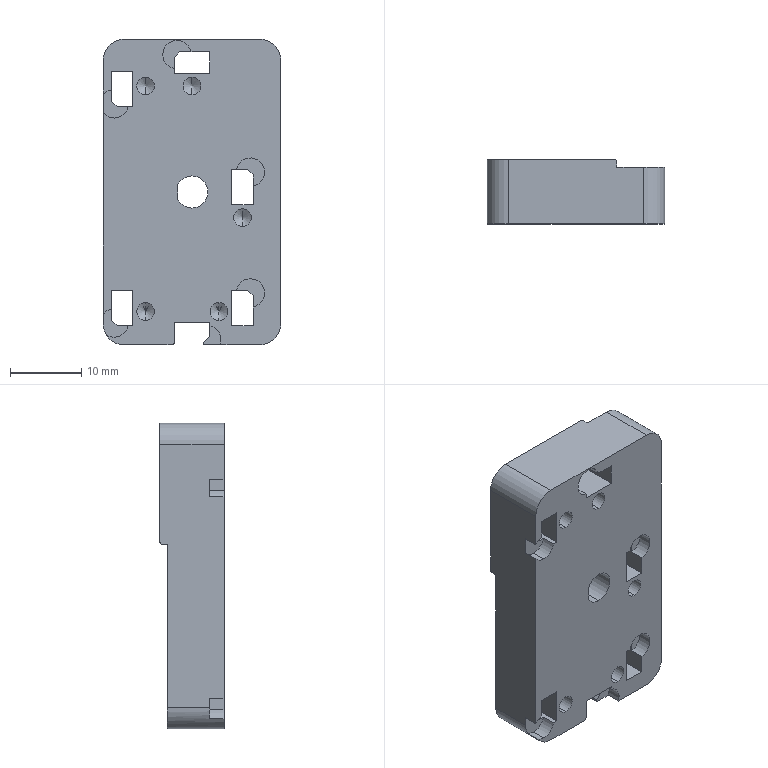Component | SolidWorks | 04LowerMaterialReceivingSwingAngleAssembly(3920)-1_04LowerMaterialReceivingDieAssembly(3920)-1_H2020022-0447-1(3920)-1 | 1 solid | 94 faces | volume 7630 mm3 | plane 47 | cylinder 34 | cone 12 | torus 1 | commonest cylinder face diameters 2.5 x10 4 x10 6 x5 4.5 x3 0.6 x3 6.5 x2 0.4 x1 | material 45#Steel